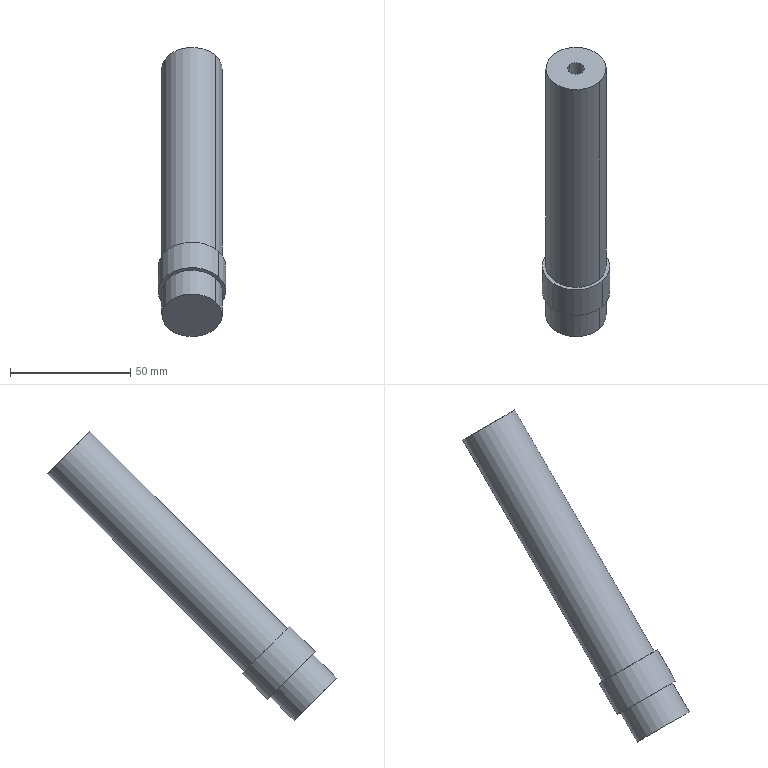Component | SolidWorks | PassiveRollerAssembly-1_SupportRollerAxis-1 | 1 solid | 14 faces | box 28 x 120.21 x 120.21 mm | volume 72308 mm3 | cylinder 8 | plane 4 | cone 2 | commonest cylinder face diameters 25 x4 6.8 x2 28 x2
build123d program:
from build123d import *

# Parameters (mm, degrees)
M8_TAPPED_HOLE1_D     = 6.8
M8_TAPPED_HOLE1_DEPTH = 19.75
M8_TAPPED_HOLE1_TIP   = 2.043


with BuildPart() as part:
    # Sketch1 → Revolve1 (revolve)
    with BuildSketch(Plane.XY, mode=Mode.PRIVATE) as revolve1_sk:
        Polygon((0, 0), (0, 12.5), (14, 12.5), (14, 14), (29, 14), (29, 12.5), (145, 12.5), (145, 0), align=None)
    revolve(revolve1_sk.sketch.rotate(Axis((-77.306, 0, 0), (1, 0, 0)), 90), axis=Axis((-77.306, 0, 0), (1, 0, 0)))

    # M8 Tapped Hole1
    with Locations(Plane(origin=(145, 0, 0), x_dir=(0, 0, -1), z_dir=(1, 0, 0))):
        with Locations((0, 0)):
            Hole(M8_TAPPED_HOLE1_D / 2, depth=M8_TAPPED_HOLE1_DEPTH)
            with Locations((0, 0, -(M8_TAPPED_HOLE1_DEPTH + M8_TAPPED_HOLE1_TIP / 2))):  # 118° drill point
                Cone(0, M8_TAPPED_HOLE1_D / 2, M8_TAPPED_HOLE1_TIP, mode=Mode.SUBTRACT)


solid = part.part

# Placed as in the assembly
solid = solid.moved(Location((2216.026, 645.044, 278.657), (-135, -21.484, -90)))
STEP:
#1=COLOUR_RGB('',0.7922,0.8196,0.9333);
#2=FILL_AREA_STYLE_COLOUR('',#1);
#3=FILL_AREA_STYLE('',(#2));
#4=SURFACE_STYLE_FILL_AREA(#3);
#5=SURFACE_SIDE_STYLE('',(#4));
#6=SURFACE_STYLE_USAGE(.BOTH.,#5);
#7=PRESENTATION_STYLE_ASSIGNMENT((#6));
#8=CARTESIAN_POINT('',(87.35,28.823,14.517));
#9=VERTEX_POINT('',#8);
#10=CARTESIAN_POINT('',(87.141,28.941,14.398));
#11=VERTEX_POINT('',#10);
#12=CARTESIAN_POINT('',(87.245,28.882,14.458));
#13=DIRECTION('',(-0.,0.7071,0.7071));
#14=DIRECTION('',(-0.7805,0.4421,-0.4421));
#15=AXIS2_PLACEMENT_3D('',#12,#13,#14);
#16=CIRCLE('',#15,0.1339);
#17=EDGE_CURVE('',#9,#11,#16,.T.);
#18=ORIENTED_EDGE('',*,*,#17,.F.);
#19=CARTESIAN_POINT('',(87.35,29.373,15.067));
#20=VERTEX_POINT('',#19);
#21=CARTESIAN_POINT('',(87.35,29.373,15.067));
#22=DIRECTION('',(-0.,0.7071,0.7071));
#23=VECTOR('',#22,39.37);
#24=LINE('',#21,#23);
#25=EDGE_CURVE('',#9,#20,#24,.T.);
#26=ORIENTED_EDGE('',*,*,#25,.T.);
#27=CARTESIAN_POINT('',(87.141,29.491,14.948));
#28=VERTEX_POINT('',#27);
#29=CARTESIAN_POINT('',(87.245,29.432,15.007));
#30=DIRECTION('',(-0.,0.7071,0.7071));
#31=DIRECTION('',(-0.7805,0.4421,-0.4421));
#32=AXIS2_PLACEMENT_3D('',#29,#30,#31);
#33=CIRCLE('',#32,0.1339);
#34=EDGE_CURVE('',#20,#28,#33,.T.);
#35=ORIENTED_EDGE('',*,*,#34,.T.);
#36=CARTESIAN_POINT('',(87.141,29.491,14.948));
#37=DIRECTION('',(-0.,0.7071,0.7071));
#38=VECTOR('',#37,39.37);
#39=LINE('',#36,#38);
#40=EDGE_CURVE('',#11,#28,#39,.T.);
#41=ORIENTED_EDGE('',*,*,#40,.F.);
#42=EDGE_LOOP('',(#18,#26,#35,#41));
#43=FACE_OUTER_BOUND('',#42,.T.);
#44=CARTESIAN_POINT('',(87.245,29.432,15.007));
#45=DIRECTION('',(-0.,0.7071,0.7071));
#46=DIRECTION('',(-0.7805,0.4421,-0.4421));
#47=AXIS2_PLACEMENT_3D('',#44,#45,#46);
#48=CYLINDRICAL_SURFACE('',#47,0.1339);
#49=ADVANCED_FACE('',(#43),#48,.F.);
#50=CARTESIAN_POINT('',(87.245,28.825,14.401));
#51=VERTEX_POINT('',#50);
#52=CARTESIAN_POINT('',(87.141,28.941,14.398));
#53=DIRECTION('',(-0.669,0.7431,-0.01473));
#54=VECTOR('',#53,39.37);
#55=LINE('',#52,#54);
#56=EDGE_CURVE('',#51,#11,#55,.T.);
#57=ORIENTED_EDGE('',*,*,#56,.F.);
#58=CARTESIAN_POINT('',(87.35,28.823,14.517));
#59=DIRECTION('',(0.669,-0.01473,0.7431));
#60=VECTOR('',#59,39.37);
#61=LINE('',#58,#60);
#62=EDGE_CURVE('',#51,#9,#61,.T.);
#63=ORIENTED_EDGE('',*,*,#62,.T.);
#64=ORIENTED_EDGE('',*,*,#17,.T.);
#65=EDGE_LOOP('',(#57,#63,#64));
#66=FACE_OUTER_BOUND('',#65,.T.);
#67=CARTESIAN_POINT('',(87.245,28.882,14.458));
#68=DIRECTION('',(-0.,0.7071,0.7071));
#69=DIRECTION('',(-0.7805,0.4421,-0.4421));
#70=AXIS2_PLACEMENT_3D('',#67,#68,#69);
#71=CONICAL_SURFACE('',#70,0.1339,1.03);
#72=ADVANCED_FACE('',(#66),#71,.F.);
#73=CARTESIAN_POINT('',(87.629,29.215,15.225));
#74=VERTEX_POINT('',#73);
#75=CARTESIAN_POINT('',(86.861,29.65,14.79));
#76=VERTEX_POINT('',#75);
#77=CARTESIAN_POINT('',(87.245,29.432,15.007));
#78=DIRECTION('',(0.,-0.7071,-0.7071));
#79=DIRECTION('',(0.7805,-0.4421,0.4421));
#80=AXIS2_PLACEMENT_3D('',#77,#78,#79);
#81=CIRCLE('',#80,0.4921);
#82=EDGE_CURVE('',#74,#76,#81,.T.);
#83=ORIENTED_EDGE('',*,*,#82,.T.);
#84=CARTESIAN_POINT('',(86.861,26.42,11.561));
#85=VERTEX_POINT('',#84);
#86=CARTESIAN_POINT('',(86.861,23.461,8.601));
#87=DIRECTION('',(0.,-0.7071,-0.7071));
#88=VECTOR('',#87,39.37);
#89=LINE('',#86,#88);
#90=EDGE_CURVE('',#76,#85,#89,.T.);
#91=ORIENTED_EDGE('',*,*,#90,.T.);
#92=CARTESIAN_POINT('',(87.629,25.985,11.996));
#93=VERTEX_POINT('',#92);
#94=CARTESIAN_POINT('',(87.245,26.203,11.778));
#95=DIRECTION('',(0.,-0.7071,-0.7071));
#96=DIRECTION('',(0.7805,-0.4421,0.4421));
#97=AXIS2_PLACEMENT_3D('',#94,#95,#96);
#98=CIRCLE('',#97,0.4921);
#99=EDGE_CURVE('',#93,#85,#98,.T.);
#100=ORIENTED_EDGE('',*,*,#99,.F.);
#101=CARTESIAN_POINT('',(87.629,23.026,9.036));
#102=DIRECTION('',(0.,-0.7071,-0.7071));
#103=VECTOR('',#102,39.37);
#104=LINE('',#101,#103);
#105=EDGE_CURVE('',#74,#93,#104,.T.);
#106=ORIENTED_EDGE('',*,*,#105,.F.);
#107=EDGE_LOOP('',(#83,#91,#100,#106));
#108=FACE_OUTER_BOUND('',#107,.T.);
#109=CARTESIAN_POINT('',(87.245,23.243,8.819));
#110=DIRECTION('',(0.,-0.7071,-0.7071));
#111=DIRECTION('',(0.7805,-0.4421,0.4421));
#112=AXIS2_PLACEMENT_3D('',#109,#110,#111);
#113=CYLINDRICAL_SURFACE('',#112,0.4921);
#114=ADVANCED_FACE('',(#108),#113,.T.);
#115=CARTESIAN_POINT('',(87.675,25.959,12.022));
#116=VERTEX_POINT('',#115);
#117=CARTESIAN_POINT('',(86.815,26.446,11.534));
#118=VERTEX_POINT('',#117);
#119=CARTESIAN_POINT('',(87.245,26.203,11.778));
#120=DIRECTION('',(0.,-0.7071,-0.7071));
#121=DIRECTION('',(0.7805,-0.4421,0.4421));
#122=AXIS2_PLACEMENT_3D('',#119,#120,#121);
#123=CIRCLE('',#122,0.5512);
#124=EDGE_CURVE('',#116,#118,#123,.T.);
#125=ORIENTED_EDGE('',*,*,#124,.T.);
#126=CARTESIAN_POINT('',(86.815,26.029,11.117));
#127=VERTEX_POINT('',#126);
#128=CARTESIAN_POINT('',(86.815,23.487,8.575));
#129=DIRECTION('',(0.,-0.7071,-0.7071));
#130=VECTOR('',#129,39.37);
#131=LINE('',#128,#130);
#132=EDGE_CURVE('',#118,#127,#131,.T.);
#133=ORIENTED_EDGE('',*,*,#132,.T.);
#134=CARTESIAN_POINT('',(87.675,25.542,11.604));
#135=VERTEX_POINT('',#134);
#136=CARTESIAN_POINT('',(87.245,25.785,11.36));
#137=DIRECTION('',(0.,-0.7071,-0.7071));
#138=DIRECTION('',(0.7805,-0.4421,0.4421));
#139=AXIS2_PLACEMENT_3D('',#136,#137,#138);
#140=CIRCLE('',#139,0.5512);
#141=EDGE_CURVE('',#135,#127,#140,.T.);
#142=ORIENTED_EDGE('',*,*,#141,.F.);
#143=CARTESIAN_POINT('',(87.675,23.,9.062));
#144=DIRECTION('',(0.,-0.7071,-0.7071));
#145=VECTOR('',#144,39.37);
#146=LINE('',#143,#145);
#147=EDGE_CURVE('',#116,#135,#146,.T.);
#148=ORIENTED_EDGE('',*,*,#147,.F.);
#149=EDGE_LOOP('',(#125,#133,#142,#148));
#150=FACE_OUTER_BOUND('',#149,.T.);
#151=CARTESIAN_POINT('',(87.245,23.243,8.819));
#152=DIRECTION('',(0.,-0.7071,-0.7071));
#153=DIRECTION('',(0.7805,-0.4421,0.4421));
#154=AXIS2_PLACEMENT_3D('',#151,#152,#153);
#155=CYLINDRICAL_SURFACE('',#154,0.5512);
#156=ADVANCED_FACE('',(#150),#155,.T.);
#157=CARTESIAN_POINT('',(87.629,25.568,11.578));
#158=VERTEX_POINT('',#157);
#159=CARTESIAN_POINT('',(86.861,26.003,11.143));
#160=VERTEX_POINT('',#159);
#161=CARTESIAN_POINT('',(87.245,25.785,11.36));
#162=DIRECTION('',(0.,-0.7071,-0.7071));
#163=DIRECTION('',(0.7805,-0.4421,0.4421));
#164=AXIS2_PLACEMENT_3D('',#161,#162,#163);
#165=CIRCLE('',#164,0.4921);
#166=EDGE_CURVE('',#158,#160,#165,.T.);
#167=ORIENTED_EDGE('',*,*,#166,.T.);
#168=CARTESIAN_POINT('',(86.861,25.613,10.753));
#169=VERTEX_POINT('',#168);
#170=CARTESIAN_POINT('',(86.861,23.461,8.601));
#171=DIRECTION('',(0.,-0.7071,-0.7071));
#172=VECTOR('',#171,39.37);
#173=LINE('',#170,#172);
#174=EDGE_CURVE('',#160,#169,#173,.T.);
#175=ORIENTED_EDGE('',*,*,#174,.T.);
#176=CARTESIAN_POINT('',(87.629,25.178,11.188));
#177=VERTEX_POINT('',#176);
#178=CARTESIAN_POINT('',(87.245,25.395,10.971));
#179=DIRECTION('',(0.,-0.7071,-0.7071));
#180=DIRECTION('',(0.7805,-0.4421,0.4421));
#181=AXIS2_PLACEMENT_3D('',#178,#179,#180);
#182=CIRCLE('',#181,0.4921);
#183=EDGE_CURVE('',#177,#169,#182,.T.);
#184=ORIENTED_EDGE('',*,*,#183,.F.);
#185=CARTESIAN_POINT('',(87.629,23.026,9.036));
#186=DIRECTION('',(0.,-0.7071,-0.7071));
#187=VECTOR('',#186,39.37);
#188=LINE('',#185,#187);
#189=EDGE_CURVE('',#158,#177,#188,.T.);
#190=ORIENTED_EDGE('',*,*,#189,.F.);
#191=EDGE_LOOP('',(#167,#175,#184,#190));
#192=FACE_OUTER_BOUND('',#191,.T.);
#193=CARTESIAN_POINT('',(87.245,23.243,8.819));
#194=DIRECTION('',(0.,-0.7071,-0.7071));
#195=DIRECTION('',(0.7805,-0.4421,0.4421));
#196=AXIS2_PLACEMENT_3D('',#193,#194,#195);
#197=CYLINDRICAL_SURFACE('',#196,0.4921);
#198=ADVANCED_FACE('',(#192),#197,.T.);
#199=ORIENTED_EDGE('',*,*,#183,.T.);
#200=CARTESIAN_POINT('',(87.245,25.395,10.971));
#201=DIRECTION('',(0.,-0.7071,-0.7071));
#202=DIRECTION('',(0.7805,-0.4421,0.4421));
#203=AXIS2_PLACEMENT_3D('',#200,#201,#202);
#204=CIRCLE('',#203,0.4921);
#205=EDGE_CURVE('',#169,#177,#204,.T.);
#206=ORIENTED_EDGE('',*,*,#205,.T.);
#207=EDGE_LOOP('',(#199,#206));
#208=FACE_OUTER_BOUND('',#207,.T.);
#209=CARTESIAN_POINT('',(87.245,25.395,10.971));
#210=DIRECTION('',(-0.,0.7071,0.7071));
#211=DIRECTION('',(-0.7805,0.4421,-0.4421));
#212=AXIS2_PLACEMENT_3D('',#209,#210,#211);
#213=PLANE('',#212);
#214=ADVANCED_FACE('',(#208),#213,.F.);
#215=ORIENTED_EDGE('',*,*,#174,.F.);
#216=CARTESIAN_POINT('',(87.245,25.785,11.36));
#217=DIRECTION('',(0.,-0.7071,-0.7071));
#218=DIRECTION('',(0.7805,-0.4421,0.4421));
#219=AXIS2_PLACEMENT_3D('',#216,#217,#218);
#220=CIRCLE('',#219,0.4921);
#221=EDGE_CURVE('',#160,#158,#220,.T.);
#222=ORIENTED_EDGE('',*,*,#221,.T.);
#223=ORIENTED_EDGE('',*,*,#189,.T.);
#224=ORIENTED_EDGE('',*,*,#205,.F.);
#225=EDGE_LOOP('',(#215,#222,#223,#224));
#226=FACE_OUTER_BOUND('',#225,.T.);
#227=CARTESIAN_POINT('',(87.245,23.243,8.819));
#228=DIRECTION('',(0.,-0.7071,-0.7071));
#229=DIRECTION('',(0.7805,-0.4421,0.4421));
#230=AXIS2_PLACEMENT_3D('',#227,#228,#229);
#231=CYLINDRICAL_SURFACE('',#230,0.4921);
#232=ADVANCED_FACE('',(#226),#231,.T.);
#233=ORIENTED_EDGE('',*,*,#166,.F.);
#234=ORIENTED_EDGE('',*,*,#221,.F.);
#235=EDGE_LOOP('',(#233,#234));
#236=FACE_BOUND('',#235,.T.);
#237=ORIENTED_EDGE('',*,*,#141,.T.);
#238=CARTESIAN_POINT('',(87.245,25.785,11.36));
#239=DIRECTION('',(0.,-0.7071,-0.7071));
#240=DIRECTION('',(0.7805,-0.4421,0.4421));
#241=AXIS2_PLACEMENT_3D('',#238,#239,#240);
#242=CIRCLE('',#241,0.5512);
#243=EDGE_CURVE('',#127,#135,#242,.T.);
#244=ORIENTED_EDGE('',*,*,#243,.T.);
#245=EDGE_LOOP('',(#237,#244));
#246=FACE_OUTER_BOUND('',#245,.T.);
#247=CARTESIAN_POINT('',(86.937,25.514,11.632));
#248=DIRECTION('',(-0.,0.7071,0.7071));
#249=DIRECTION('',(-0.7805,0.4421,-0.4421));
#250=AXIS2_PLACEMENT_3D('',#247,#248,#249);
#251=PLANE('',#250);
#252=ADVANCED_FACE('',(#236,#246),#251,.F.);
#253=ORIENTED_EDGE('',*,*,#132,.F.);
#254=CARTESIAN_POINT('',(87.245,26.203,11.778));
#255=DIRECTION('',(0.,-0.7071,-0.7071));
#256=DIRECTION('',(0.7805,-0.4421,0.4421));
#257=AXIS2_PLACEMENT_3D('',#254,#255,#256);
#258=CIRCLE('',#257,0.5512);
#259=EDGE_CURVE('',#118,#116,#258,.T.);
#260=ORIENTED_EDGE('',*,*,#259,.T.);
#261=ORIENTED_EDGE('',*,*,#147,.T.);
#262=ORIENTED_EDGE('',*,*,#243,.F.);
#263=EDGE_LOOP('',(#253,#260,#261,#262));
#264=FACE_OUTER_BOUND('',#263,.T.);
#265=CARTESIAN_POINT('',(87.245,23.243,8.819));
#266=DIRECTION('',(0.,-0.7071,-0.7071));
#267=DIRECTION('',(0.7805,-0.4421,0.4421));
#268=AXIS2_PLACEMENT_3D('',#265,#266,#267);
#269=CYLINDRICAL_SURFACE('',#268,0.5512);
#270=ADVANCED_FACE('',(#264),#269,.T.);
#271=ORIENTED_EDGE('',*,*,#124,.F.);
#272=ORIENTED_EDGE('',*,*,#259,.F.);
#273=EDGE_LOOP('',(#271,#272));
#274=FACE_OUTER_BOUND('',#273,.T.);
#275=ORIENTED_EDGE('',*,*,#99,.T.);
#276=CARTESIAN_POINT('',(87.245,26.203,11.778));
#277=DIRECTION('',(0.,-0.7071,-0.7071));
#278=DIRECTION('',(0.7805,-0.4421,0.4421));
#279=AXIS2_PLACEMENT_3D('',#276,#277,#278);
#280=CIRCLE('',#279,0.4921);
#281=EDGE_CURVE('',#85,#93,#280,.T.);
#282=ORIENTED_EDGE('',*,*,#281,.T.);
#283=EDGE_LOOP('',(#275,#282));
#284=FACE_BOUND('',#283,.T.);
#285=CARTESIAN_POINT('',(86.901,25.899,12.082));
#286=DIRECTION('',(0.,-0.7071,-0.7071));
#287=DIRECTION('',(0.7805,-0.4421,0.4421));
#288=AXIS2_PLACEMENT_3D('',#285,#286,#287);
#289=PLANE('',#288);
#290=ADVANCED_FACE('',(#274,#284),#289,.F.);
#291=ORIENTED_EDGE('',*,*,#90,.F.);
#292=CARTESIAN_POINT('',(87.245,29.432,15.007));
#293=DIRECTION('',(0.,-0.7071,-0.7071));
#294=DIRECTION('',(0.7805,-0.4421,0.4421));
#295=AXIS2_PLACEMENT_3D('',#292,#293,#294);
#296=CIRCLE('',#295,0.4921);
#297=EDGE_CURVE('',#76,#74,#296,.T.);
#298=ORIENTED_EDGE('',*,*,#297,.T.);
#299=ORIENTED_EDGE('',*,*,#105,.T.);
#300=ORIENTED_EDGE('',*,*,#281,.F.);
#301=EDGE_LOOP('',(#291,#298,#299,#300));
#302=FACE_OUTER_BOUND('',#301,.T.);
#303=CARTESIAN_POINT('',(87.245,23.243,8.819));
#304=DIRECTION('',(0.,-0.7071,-0.7071));
#305=DIRECTION('',(0.7805,-0.4421,0.4421));
#306=AXIS2_PLACEMENT_3D('',#303,#304,#305);
#307=CYLINDRICAL_SURFACE('',#306,0.4921);
#308=ADVANCED_FACE('',(#302),#307,.T.);
#309=CARTESIAN_POINT('',(87.245,29.432,15.007));
#310=DIRECTION('',(-0.,0.7071,0.7071));
#311=DIRECTION('',(-0.7805,0.4421,-0.4421));
#312=AXIS2_PLACEMENT_3D('',#309,#310,#311);
#313=CIRCLE('',#312,0.1339);
#314=EDGE_CURVE('',#28,#20,#313,.T.);
#315=ORIENTED_EDGE('',*,*,#314,.F.);
#316=ORIENTED_EDGE('',*,*,#34,.F.);
#317=EDGE_LOOP('',(#315,#316));
#318=FACE_BOUND('',#317,.T.);
#319=ORIENTED_EDGE('',*,*,#82,.F.);
#320=ORIENTED_EDGE('',*,*,#297,.F.);
#321=EDGE_LOOP('',(#319,#320));
#322=FACE_OUTER_BOUND('',#321,.T.);
#323=CARTESIAN_POINT('',(86.937,29.16,15.279));
#324=DIRECTION('',(0.,-0.7071,-0.7071));
#325=DIRECTION('',(0.7805,-0.4421,0.4421));
#326=AXIS2_PLACEMENT_3D('',#323,#324,#325);
#327=PLANE('',#326);
#328=ADVANCED_FACE('',(#318,#322),#327,.F.);
#329=ORIENTED_EDGE('',*,*,#62,.F.);
#330=ORIENTED_EDGE('',*,*,#56,.T.);
#331=CARTESIAN_POINT('',(87.245,28.882,14.458));
#332=DIRECTION('',(-0.,0.7071,0.7071));
#333=DIRECTION('',(-0.7805,0.4421,-0.4421));
#334=AXIS2_PLACEMENT_3D('',#331,#332,#333);
#335=CIRCLE('',#334,0.1339);
#336=EDGE_CURVE('',#11,#9,#335,.T.);
#337=ORIENTED_EDGE('',*,*,#336,.T.);
#338=EDGE_LOOP('',(#329,#330,#337));
#339=FACE_OUTER_BOUND('',#338,.T.);
#340=CARTESIAN_POINT('',(87.245,28.882,14.458));
#341=DIRECTION('',(-0.,0.7071,0.7071));
#342=DIRECTION('',(-0.7805,0.4421,-0.4421));
#343=AXIS2_PLACEMENT_3D('',#340,#341,#342);
#344=CONICAL_SURFACE('',#343,0.1339,1.03);
#345=ADVANCED_FACE('',(#339),#344,.F.);
#346=ORIENTED_EDGE('',*,*,#25,.F.);
#347=ORIENTED_EDGE('',*,*,#336,.F.);
#348=ORIENTED_EDGE('',*,*,#40,.T.);
#349=ORIENTED_EDGE('',*,*,#314,.T.);
#350=EDGE_LOOP('',(#346,#347,#348,#349));
#351=FACE_OUTER_BOUND('',#350,.T.);
#352=CARTESIAN_POINT('',(87.245,29.432,15.007));
#353=DIRECTION('',(-0.,0.7071,0.7071));
#354=DIRECTION('',(-0.7805,0.4421,-0.4421));
#355=AXIS2_PLACEMENT_3D('',#352,#353,#354);
#356=CYLINDRICAL_SURFACE('',#355,0.1339);
#357=ADVANCED_FACE('',(#351),#356,.F.);
#358=CLOSED_SHELL('',(#49,#72,#114,#156,#198,#214,#232,#252,#270,#290,#308,#328,#345,#357));
#359=MANIFOLD_SOLID_BREP('',#358);
#360=STYLED_ITEM('',(#7),#359);
#361=PRESENTATION_LAYER_ASSIGNMENT('','',(#360));
#362=CARTESIAN_POINT('',(0.,0.,0.));
#363=DIRECTION('',(0.,0.,1.));
#364=DIRECTION('',(1.,0.,0.));
#365=AXIS2_PLACEMENT_3D('',#362,#363,#364);
#366=(LENGTH_UNIT()NAMED_UNIT(*)SI_UNIT($,.METRE.));
#367=LENGTH_MEASURE_WITH_UNIT(LENGTH_MEASURE(0.0254),#366);
#368=DIMENSIONAL_EXPONENTS(1.,0.,0.,0.,0.,0.,0.);
#369=(CONVERSION_BASED_UNIT('',#367)LENGTH_UNIT()NAMED_UNIT(#368));
#370=UNCERTAINTY_MEASURE_WITH_UNIT(LENGTH_MEASURE(0.00001),#369,'','');
#371=(NAMED_UNIT(*)PLANE_ANGLE_UNIT()SI_UNIT($,.RADIAN.));
#372=(NAMED_UNIT(*)SI_UNIT($,.STERADIAN.)SOLID_ANGLE_UNIT());
#373=(GEOMETRIC_REPRESENTATION_CONTEXT(3)GLOBAL_UNCERTAINTY_ASSIGNED_CONTEXT((#370))GLOBAL_UNIT_ASSIGNED_CONTEXT((#369,#371,#372))REPRESENTATION_CONTEXT('',''));
#374=ADVANCED_BREP_SHAPE_REPRESENTATION('',(#359,#365),#373);
#375=(LENGTH_UNIT()NAMED_UNIT(*)SI_UNIT($,.METRE.));
#376=LENGTH_MEASURE_WITH_UNIT(LENGTH_MEASURE(0.0254),#375);
#377=DIMENSIONAL_EXPONENTS(1.,0.,0.,0.,0.,0.,0.);
#378=(CONVERSION_BASED_UNIT('',#376)LENGTH_UNIT()NAMED_UNIT(#377));
#379=UNCERTAINTY_MEASURE_WITH_UNIT(LENGTH_MEASURE(0.00001),#378,'','');
#380=(NAMED_UNIT(*)PLANE_ANGLE_UNIT()SI_UNIT($,.RADIAN.));
#381=(NAMED_UNIT(*)SI_UNIT($,.STERADIAN.)SOLID_ANGLE_UNIT());
#382=(GEOMETRIC_REPRESENTATION_CONTEXT(3)GLOBAL_UNCERTAINTY_ASSIGNED_CONTEXT((#379))GLOBAL_UNIT_ASSIGNED_CONTEXT((#378,#380,#381))REPRESENTATION_CONTEXT('',''));
#383=MECHANICAL_DESIGN_GEOMETRIC_PRESENTATION_REPRESENTATION('',(#360),#382);